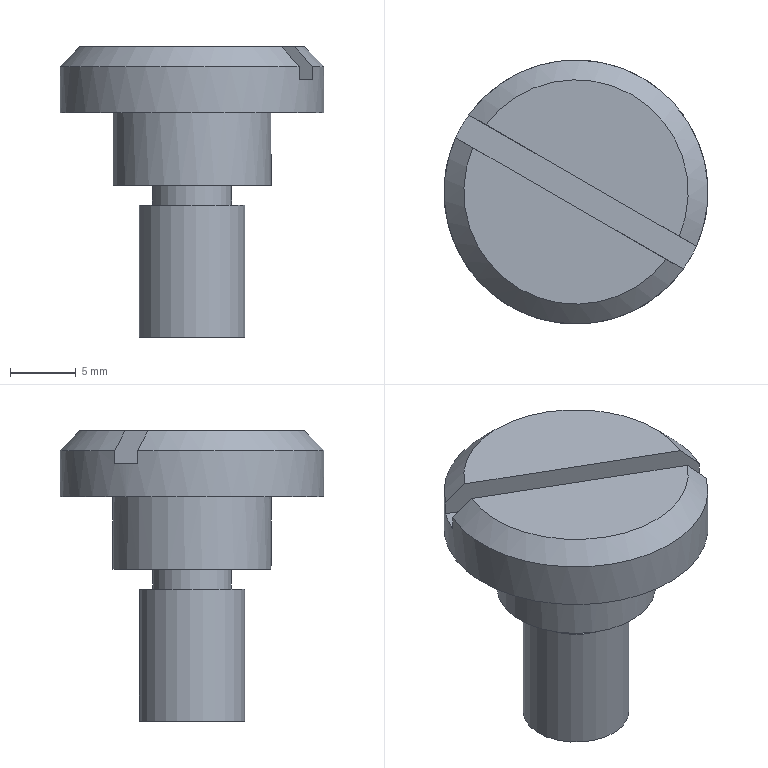Component | NX | DRILL_BUSH_SCREW | 1 solid | 15 faces | box 20 x 20 x 22 mm | volume 2575 mm3 | plane 9 | cylinder 4 | cone 2 | commonest cylinder face diameters 8 x1 6 x1 12 x1 20 x1
STEP:
#1=CARTESIAN_POINT('',(0.,0.,0.));
#2=DIRECTION('',(0.,0.,1.));
#3=DIRECTION('',(1.,0.,0.));
#4=AXIS2_PLACEMENT_3D('',#1,#2,#3);
#5=CARTESIAN_POINT('',(-19.19,-50.12,210.5));
#6=VERTEX_POINT('',#5);
#7=CARTESIAN_POINT('',(-33.81,-41.679,210.5));
#8=VERTEX_POINT('',#7);
#9=CARTESIAN_POINT('',(-13.077,-53.649,210.5));
#10=DIRECTION('',(-0.866,0.5,0.));
#11=VECTOR('',#10,1.);
#12=LINE('',#9,#11);
#13=CARTESIAN_POINT('',(-27.,-46.765,210.5));
#14=DIRECTION('',(0.,0.,1.));
#15=DIRECTION('',(-0.866,0.5,0.));
#16=AXIS2_PLACEMENT_3D('',#13,#14,#15);
#17=PLANE('',#16);
#18=CARTESIAN_POINT('',(-15.5,-1.));
#19=DIRECTION('',(1.,0.));
#20=VECTOR('',#19,1.);
#21=LINE('',#18,#20);
#22=(GEOMETRIC_REPRESENTATION_CONTEXT(2)PARAMETRIC_REPRESENTATION_CONTEXT()REPRESENTATION_CONTEXT('',''));
#23=DEFINITIONAL_REPRESENTATION('',(#21),#22);
#24=PCURVE('',#17,#23);
#25=CARTESIAN_POINT('',(-13.077,-53.649,208.));
#26=DIRECTION('',(0.5,0.866,0.));
#27=DIRECTION('',(0.,0.,-1.));
#28=AXIS2_PLACEMENT_3D('',#25,#26,#27);
#29=PLANE('',#28);
#30=CARTESIAN_POINT('',(-2.5,0.));
#31=DIRECTION('',(0.,1.));
#32=VECTOR('',#31,1.);
#33=LINE('',#30,#32);
#34=(GEOMETRIC_REPRESENTATION_CONTEXT(2)PARAMETRIC_REPRESENTATION_CONTEXT()REPRESENTATION_CONTEXT('',''));
#35=DEFINITIONAL_REPRESENTATION('',(#33),#34);
#36=PCURVE('',#29,#35);
#37=SURFACE_CURVE('',#12,(#24,#36),.PCURVE_S1.);
#38=EDGE_CURVE('',#6,#8,#37,.T.);
#39=ORIENTED_EDGE('',*,*,#38,.F.);
#40=CARTESIAN_POINT('',(-27.,-46.765,210.5));
#41=DIRECTION('',(0.,0.,1.));
#42=DIRECTION('',(-0.866,0.5,0.));
#43=AXIS2_PLACEMENT_3D('',#40,#41,#42);
#44=CIRCLE('',#43,8.5);
#45=CARTESIAN_POINT('',(0.,0.));
#46=DIRECTION('',(1.,0.));
#47=AXIS2_PLACEMENT_2D('',#45,#46);
#48=CIRCLE('',#47,8.5);
#49=(GEOMETRIC_REPRESENTATION_CONTEXT(2)PARAMETRIC_REPRESENTATION_CONTEXT()REPRESENTATION_CONTEXT('',''));
#50=DEFINITIONAL_REPRESENTATION('',(#48),#49);
#51=PCURVE('',#17,#50);
#52=CARTESIAN_POINT('',(-27.,-46.765,209.));
#53=DIRECTION('',(0.,0.,-1.));
#54=DIRECTION('',(0.866,-0.5,0.));
#55=AXIS2_PLACEMENT_3D('',#52,#53,#54);
#56=CONICAL_SURFACE('',#55,10.,0.7854);
#57=CARTESIAN_POINT('',(9.425,-1.5));
#58=DIRECTION('',(-1.,-0.));
#59=VECTOR('',#58,1.);
#60=LINE('',#57,#59);
#61=(GEOMETRIC_REPRESENTATION_CONTEXT(2)PARAMETRIC_REPRESENTATION_CONTEXT()REPRESENTATION_CONTEXT('',''));
#62=DEFINITIONAL_REPRESENTATION('',(#60),#61);
#63=PCURVE('',#56,#62);
#64=SURFACE_CURVE('',#44,(#51,#63),.PCURVE_S1.);
#65=EDGE_CURVE('',#6,#8,#64,.T.);
#66=ORIENTED_EDGE('',*,*,#65,.T.);
#67=EDGE_LOOP('',(#39,#66));
#68=FACE_BOUND('',#67,.T.);
#69=ADVANCED_FACE('',(#68),#17,.T.);
#70=CARTESIAN_POINT('',(-29.598,-45.265,198.5));
#71=VERTEX_POINT('',#70);
#72=CARTESIAN_POINT('',(-27.,-46.765,198.5));
#73=DIRECTION('',(0.,0.,1.));
#74=DIRECTION('',(-0.866,0.5,0.));
#75=AXIS2_PLACEMENT_3D('',#72,#73,#74);
#76=CIRCLE('',#75,3.);
#77=CARTESIAN_POINT('',(-27.,-46.765,198.5));
#78=DIRECTION('',(0.,0.,1.));
#79=DIRECTION('',(-0.866,0.5,0.));
#80=AXIS2_PLACEMENT_3D('',#77,#78,#79);
#81=PLANE('',#80);
#82=CARTESIAN_POINT('',(0.,0.));
#83=DIRECTION('',(1.,-0.));
#84=AXIS2_PLACEMENT_2D('',#82,#83);
#85=CIRCLE('',#84,3.);
#86=(GEOMETRIC_REPRESENTATION_CONTEXT(2)PARAMETRIC_REPRESENTATION_CONTEXT()REPRESENTATION_CONTEXT('',''));
#87=DEFINITIONAL_REPRESENTATION('',(#85),#86);
#88=PCURVE('',#81,#87);
#89=CARTESIAN_POINT('',(-27.,-46.765,198.5));
#90=DIRECTION('',(0.,0.,1.));
#91=DIRECTION('',(-0.866,0.5,0.));
#92=AXIS2_PLACEMENT_3D('',#89,#90,#91);
#93=CYLINDRICAL_SURFACE('',#92,3.);
#94=CARTESIAN_POINT('',(0.,0.));
#95=DIRECTION('',(1.,0.));
#96=VECTOR('',#95,1.);
#97=LINE('',#94,#96);
#98=(GEOMETRIC_REPRESENTATION_CONTEXT(2)PARAMETRIC_REPRESENTATION_CONTEXT()REPRESENTATION_CONTEXT('',''));
#99=DEFINITIONAL_REPRESENTATION('',(#97),#98);
#100=PCURVE('',#93,#99);
#101=SURFACE_CURVE('',#76,(#88,#100),.PCURVE_S1.);
#102=EDGE_CURVE('',#71,#71,#101,.T.);
#103=ORIENTED_EDGE('',*,*,#102,.F.);
#104=EDGE_LOOP('',(#103));
#105=FACE_BOUND('',#104,.T.);
#106=CARTESIAN_POINT('',(-30.464,-44.765,198.5));
#107=VERTEX_POINT('',#106);
#108=CARTESIAN_POINT('',(-27.,-46.765,198.5));
#109=DIRECTION('',(0.,0.,-1.));
#110=DIRECTION('',(-0.866,0.5,0.));
#111=AXIS2_PLACEMENT_3D('',#108,#109,#110);
#112=CIRCLE('',#111,4.);
#113=CARTESIAN_POINT('',(4.,-0.));
#114=CARTESIAN_POINT('',(4.,-6.928));
#115=CARTESIAN_POINT('',(-2.,-3.464));
#116=CARTESIAN_POINT('',(-8.,0.));
#117=CARTESIAN_POINT('',(-2.,3.464));
#118=CARTESIAN_POINT('',(4.,6.928));
#119=CARTESIAN_POINT('',(4.,-0.));
#120=(BOUNDED_CURVE()B_SPLINE_CURVE(2,(#113,#114,#115,#116,#117,#118,#119),.UNSPECIFIED.,.T.,.F.)B_SPLINE_CURVE_WITH_KNOTS((1,2,2,2,2,1),(-2.094,0.,2.094,4.189,6.283,8.378),.UNSPECIFIED.)CURVE()GEOMETRIC_REPRESENTATION_ITEM()RATIONAL_B_SPLINE_CURVE((1.,0.5,1.,0.5,1.,0.5,1.))REPRESENTATION_ITEM(''));
#121=(GEOMETRIC_REPRESENTATION_CONTEXT(2)PARAMETRIC_REPRESENTATION_CONTEXT()REPRESENTATION_CONTEXT('',''));
#122=DEFINITIONAL_REPRESENTATION('',(#120),#121);
#123=PCURVE('',#81,#122);
#124=CARTESIAN_POINT('',(-27.,-46.765,188.5));
#125=DIRECTION('',(0.,0.,1.));
#126=DIRECTION('',(-0.866,0.5,0.));
#127=AXIS2_PLACEMENT_3D('',#124,#125,#126);
#128=CYLINDRICAL_SURFACE('',#127,4.);
#129=CARTESIAN_POINT('',(6.283,10.));
#130=DIRECTION('',(-1.,0.));
#131=VECTOR('',#130,1.);
#132=LINE('',#129,#131);
#133=(GEOMETRIC_REPRESENTATION_CONTEXT(2)PARAMETRIC_REPRESENTATION_CONTEXT()REPRESENTATION_CONTEXT('',''));
#134=DEFINITIONAL_REPRESENTATION('',(#132),#133);
#135=PCURVE('',#128,#134);
#136=SURFACE_CURVE('',#112,(#123,#135),.PCURVE_S1.);
#137=EDGE_CURVE('',#107,#107,#136,.T.);
#138=ORIENTED_EDGE('',*,*,#137,.F.);
#139=EDGE_LOOP('',(#138));
#140=FACE_BOUND('',#139,.T.);
#141=ADVANCED_FACE('',(#105,#140),#81,.T.);
#142=CARTESIAN_POINT('',(-30.464,-44.765,188.5));
#143=VERTEX_POINT('',#142);
#144=CARTESIAN_POINT('',(-27.,-46.765,188.5));
#145=DIRECTION('',(0.,0.,1.));
#146=DIRECTION('',(-0.866,0.5,0.));
#147=AXIS2_PLACEMENT_3D('',#144,#145,#146);
#148=CIRCLE('',#147,4.);
#149=CARTESIAN_POINT('',(-27.,-46.765,188.5));
#150=DIRECTION('',(0.,0.,-1.));
#151=DIRECTION('',(0.866,-0.5,0.));
#152=AXIS2_PLACEMENT_3D('',#149,#150,#151);
#153=PLANE('',#152);
#154=CARTESIAN_POINT('',(-4.,-0.));
#155=CARTESIAN_POINT('',(-4.,6.928));
#156=CARTESIAN_POINT('',(2.,3.464));
#157=CARTESIAN_POINT('',(8.,0.));
#158=CARTESIAN_POINT('',(2.,-3.464));
#159=CARTESIAN_POINT('',(-4.,-6.928));
#160=CARTESIAN_POINT('',(-4.,-0.));
#161=(BOUNDED_CURVE()B_SPLINE_CURVE(2,(#154,#155,#156,#157,#158,#159,#160),.UNSPECIFIED.,.T.,.F.)B_SPLINE_CURVE_WITH_KNOTS((1,2,2,2,2,1),(-2.094,0.,2.094,4.189,6.283,8.378),.UNSPECIFIED.)CURVE()GEOMETRIC_REPRESENTATION_ITEM()RATIONAL_B_SPLINE_CURVE((1.,0.5,1.,0.5,1.,0.5,1.))REPRESENTATION_ITEM(''));
#162=(GEOMETRIC_REPRESENTATION_CONTEXT(2)PARAMETRIC_REPRESENTATION_CONTEXT()REPRESENTATION_CONTEXT('',''));
#163=DEFINITIONAL_REPRESENTATION('',(#161),#162);
#164=PCURVE('',#153,#163);
#165=CARTESIAN_POINT('',(0.,0.));
#166=DIRECTION('',(1.,0.));
#167=VECTOR('',#166,1.);
#168=LINE('',#165,#167);
#169=(GEOMETRIC_REPRESENTATION_CONTEXT(2)PARAMETRIC_REPRESENTATION_CONTEXT()REPRESENTATION_CONTEXT('',''));
#170=DEFINITIONAL_REPRESENTATION('',(#168),#169);
#171=PCURVE('',#128,#170);
#172=SURFACE_CURVE('',#148,(#164,#171),.PCURVE_S1.);
#173=EDGE_CURVE('',#143,#143,#172,.T.);
#174=ORIENTED_EDGE('',*,*,#173,.F.);
#175=EDGE_LOOP('',(#174));
#176=FACE_BOUND('',#175,.T.);
#177=ADVANCED_FACE('',(#176),#153,.T.);
#178=ORIENTED_EDGE('',*,*,#137,.T.);
#179=CARTESIAN_POINT('',(-30.464,-44.765,188.5));
#180=CARTESIAN_POINT('',(-30.464,-44.765,198.5));
#181=B_SPLINE_CURVE_WITH_KNOTS('',1,(#179,#180),.UNSPECIFIED.,.F.,.F.,(2,2),(0.,10.),.PIECEWISE_BEZIER_KNOTS.);
#182=CARTESIAN_POINT('',(0.,0.));
#183=DIRECTION('',(0.,1.));
#184=VECTOR('',#183,1.);
#185=LINE('',#182,#184);
#186=(GEOMETRIC_REPRESENTATION_CONTEXT(2)PARAMETRIC_REPRESENTATION_CONTEXT()REPRESENTATION_CONTEXT('',''));
#187=DEFINITIONAL_REPRESENTATION('',(#185),#186);
#188=PCURVE('',#128,#187);
#189=CARTESIAN_POINT('',(6.283,0.));
#190=DIRECTION('',(0.,1.));
#191=VECTOR('',#190,1.);
#192=LINE('',#189,#191);
#193=(GEOMETRIC_REPRESENTATION_CONTEXT(2)PARAMETRIC_REPRESENTATION_CONTEXT()REPRESENTATION_CONTEXT('',''));
#194=DEFINITIONAL_REPRESENTATION('',(#192),#193);
#195=PCURVE('',#128,#194);
#196=SEAM_CURVE('',#181,(#188,#195),.PCURVE_S1.);
#197=EDGE_CURVE('',#143,#107,#196,.T.);
#198=ORIENTED_EDGE('',*,*,#197,.F.);
#199=ORIENTED_EDGE('',*,*,#173,.T.);
#200=ORIENTED_EDGE('',*,*,#197,.T.);
#201=EDGE_LOOP('',(#178,#198,#199,#200));
#202=FACE_BOUND('',#201,.T.);
#203=ADVANCED_FACE('',(#202),#128,.T.);
#204=CARTESIAN_POINT('',(-29.598,-45.265,200.));
#205=VERTEX_POINT('',#204);
#206=CARTESIAN_POINT('',(-24.402,-48.265,200.));
#207=VERTEX_POINT('',#206);
#208=CARTESIAN_POINT('',(-27.,-46.765,200.));
#209=DIRECTION('',(0.,0.,1.));
#210=DIRECTION('',(0.866,-0.5,0.));
#211=AXIS2_PLACEMENT_3D('',#208,#209,#210);
#212=CIRCLE('',#211,3.);
#213=CARTESIAN_POINT('',(-3.142,1.5));
#214=DIRECTION('',(1.,0.));
#215=VECTOR('',#214,1.);
#216=LINE('',#213,#215);
#217=(GEOMETRIC_REPRESENTATION_CONTEXT(2)PARAMETRIC_REPRESENTATION_CONTEXT()REPRESENTATION_CONTEXT('',''));
#218=DEFINITIONAL_REPRESENTATION('',(#216),#217);
#219=PCURVE('',#93,#218);
#220=CARTESIAN_POINT('',(-27.,-46.765,200.));
#221=DIRECTION('',(0.,0.,-1.));
#222=DIRECTION('',(0.866,-0.5,0.));
#223=AXIS2_PLACEMENT_3D('',#220,#221,#222);
#224=PLANE('',#223);
#225=CARTESIAN_POINT('',(3.,0.));
#226=CARTESIAN_POINT('',(3.,-5.196));
#227=CARTESIAN_POINT('',(-1.5,-2.598));
#228=CARTESIAN_POINT('',(-6.,-0.));
#229=CARTESIAN_POINT('',(-1.5,2.598));
#230=CARTESIAN_POINT('',(3.,5.196));
#231=CARTESIAN_POINT('',(3.,0.));
#232=(BOUNDED_CURVE()B_SPLINE_CURVE(2,(#225,#226,#227,#228,#229,#230,#231),.UNSPECIFIED.,.T.,.F.)B_SPLINE_CURVE_WITH_KNOTS((1,2,2,2,2,1),(-2.094,0.,2.094,4.189,6.283,8.378),.UNSPECIFIED.)CURVE()GEOMETRIC_REPRESENTATION_ITEM()RATIONAL_B_SPLINE_CURVE((1.,0.5,1.,0.5,1.,0.5,1.))REPRESENTATION_ITEM(''));
#233=(GEOMETRIC_REPRESENTATION_CONTEXT(2)PARAMETRIC_REPRESENTATION_CONTEXT()REPRESENTATION_CONTEXT('',''));
#234=DEFINITIONAL_REPRESENTATION('',(#232),#233);
#235=PCURVE('',#224,#234);
#236=SURFACE_CURVE('',#212,(#219,#235),.PCURVE_S1.);
#237=EDGE_CURVE('',#205,#207,#236,.T.);
#238=ORIENTED_EDGE('',*,*,#237,.F.);
#239=CARTESIAN_POINT('',(-29.598,-45.265,198.5));
#240=CARTESIAN_POINT('',(-29.598,-45.265,200.));
#241=B_SPLINE_CURVE_WITH_KNOTS('',1,(#239,#240),.UNSPECIFIED.,.F.,.F.,(2,2),(0.,1.5),.PIECEWISE_BEZIER_KNOTS.);
#242=CARTESIAN_POINT('',(0.,0.));
#243=DIRECTION('',(0.,1.));
#244=VECTOR('',#243,1.);
#245=LINE('',#242,#244);
#246=(GEOMETRIC_REPRESENTATION_CONTEXT(2)PARAMETRIC_REPRESENTATION_CONTEXT()REPRESENTATION_CONTEXT('',''));
#247=DEFINITIONAL_REPRESENTATION('',(#245),#246);
#248=PCURVE('',#93,#247);
#249=CARTESIAN_POINT('',(6.283,0.));
#250=DIRECTION('',(0.,1.));
#251=VECTOR('',#250,1.);
#252=LINE('',#249,#251);
#253=(GEOMETRIC_REPRESENTATION_CONTEXT(2)PARAMETRIC_REPRESENTATION_CONTEXT()REPRESENTATION_CONTEXT('',''));
#254=DEFINITIONAL_REPRESENTATION('',(#252),#253);
#255=PCURVE('',#93,#254);
#256=SEAM_CURVE('',#241,(#248,#255),.PCURVE_S1.);
#257=EDGE_CURVE('',#71,#205,#256,.T.);
#258=ORIENTED_EDGE('',*,*,#257,.F.);
#259=ORIENTED_EDGE('',*,*,#102,.T.);
#260=ORIENTED_EDGE('',*,*,#257,.T.);
#261=CARTESIAN_POINT('',(-27.,-46.765,200.));
#262=DIRECTION('',(0.,0.,1.));
#263=DIRECTION('',(0.866,-0.5,0.));
#264=AXIS2_PLACEMENT_3D('',#261,#262,#263);
#265=CIRCLE('',#264,3.);
#266=CARTESIAN_POINT('',(3.142,1.5));
#267=DIRECTION('',(1.,0.));
#268=VECTOR('',#267,1.);
#269=LINE('',#266,#268);
#270=(GEOMETRIC_REPRESENTATION_CONTEXT(2)PARAMETRIC_REPRESENTATION_CONTEXT()REPRESENTATION_CONTEXT('',''));
#271=DEFINITIONAL_REPRESENTATION('',(#269),#270);
#272=PCURVE('',#93,#271);
#273=CARTESIAN_POINT('',(3.,0.));
#274=CARTESIAN_POINT('',(3.,-5.196));
#275=CARTESIAN_POINT('',(-1.5,-2.598));
#276=CARTESIAN_POINT('',(-6.,-0.));
#277=CARTESIAN_POINT('',(-1.5,2.598));
#278=CARTESIAN_POINT('',(3.,5.196));
#279=CARTESIAN_POINT('',(3.,0.));
#280=(BOUNDED_CURVE()B_SPLINE_CURVE(2,(#273,#274,#275,#276,#277,#278,#279),.UNSPECIFIED.,.T.,.F.)B_SPLINE_CURVE_WITH_KNOTS((1,2,2,2,2,1),(-2.094,0.,2.094,4.189,6.283,8.378),.UNSPECIFIED.)CURVE()GEOMETRIC_REPRESENTATION_ITEM()RATIONAL_B_SPLINE_CURVE((1.,0.5,1.,0.5,1.,0.5,1.))REPRESENTATION_ITEM(''));
#281=(GEOMETRIC_REPRESENTATION_CONTEXT(2)PARAMETRIC_REPRESENTATION_CONTEXT()REPRESENTATION_CONTEXT('',''));
#282=DEFINITIONAL_REPRESENTATION('',(#280),#281);
#283=PCURVE('',#224,#282);
#284=SURFACE_CURVE('',#265,(#272,#283),.PCURVE_S1.);
#285=EDGE_CURVE('',#207,#205,#284,.T.);
#286=ORIENTED_EDGE('',*,*,#285,.F.);
#287=EDGE_LOOP('',(#238,#258,#259,#260,#286));
#288=FACE_BOUND('',#287,.T.);
#289=ADVANCED_FACE('',(#288),#93,.T.);
#290=ORIENTED_EDGE('',*,*,#285,.T.);
#291=ORIENTED_EDGE('',*,*,#237,.T.);
#292=EDGE_LOOP('',(#290,#291));
#293=FACE_BOUND('',#292,.T.);
#294=CARTESIAN_POINT('',(-32.196,-43.765,200.));
#295=VERTEX_POINT('',#294);
#296=CARTESIAN_POINT('',(-27.,-46.765,200.));
#297=DIRECTION('',(0.,0.,1.));
#298=DIRECTION('',(-0.866,0.5,0.));
#299=AXIS2_PLACEMENT_3D('',#296,#297,#298);
#300=CIRCLE('',#299,6.);
#301=CARTESIAN_POINT('',(-6.,0.));
#302=CARTESIAN_POINT('',(-6.,10.392));
#303=CARTESIAN_POINT('',(3.,5.196));
#304=CARTESIAN_POINT('',(12.,0.));
#305=CARTESIAN_POINT('',(3.,-5.196));
#306=CARTESIAN_POINT('',(-6.,-10.392));
#307=CARTESIAN_POINT('',(-6.,0.));
#308=(BOUNDED_CURVE()B_SPLINE_CURVE(2,(#301,#302,#303,#304,#305,#306,#307),.UNSPECIFIED.,.T.,.F.)B_SPLINE_CURVE_WITH_KNOTS((1,2,2,2,2,1),(-2.094,0.,2.094,4.189,6.283,8.378),.UNSPECIFIED.)CURVE()GEOMETRIC_REPRESENTATION_ITEM()RATIONAL_B_SPLINE_CURVE((1.,0.5,1.,0.5,1.,0.5,1.))REPRESENTATION_ITEM(''));
#309=(GEOMETRIC_REPRESENTATION_CONTEXT(2)PARAMETRIC_REPRESENTATION_CONTEXT()REPRESENTATION_CONTEXT('',''));
#310=DEFINITIONAL_REPRESENTATION('',(#308),#309);
#311=PCURVE('',#224,#310);
#312=CARTESIAN_POINT('',(-27.,-46.765,200.));
#313=DIRECTION('',(0.,0.,1.));
#314=DIRECTION('',(-0.866,0.5,0.));
#315=AXIS2_PLACEMENT_3D('',#312,#313,#314);
#316=CYLINDRICAL_SURFACE('',#315,6.);
#317=CARTESIAN_POINT('',(0.,0.));
#318=DIRECTION('',(1.,0.));
#319=VECTOR('',#318,1.);
#320=LINE('',#317,#319);
#321=(GEOMETRIC_REPRESENTATION_CONTEXT(2)PARAMETRIC_REPRESENTATION_CONTEXT()REPRESENTATION_CONTEXT('',''));
#322=DEFINITIONAL_REPRESENTATION('',(#320),#321);
#323=PCURVE('',#316,#322);
#324=SURFACE_CURVE('',#300,(#311,#323),.PCURVE_S1.);
#325=EDGE_CURVE('',#295,#295,#324,.T.);
#326=ORIENTED_EDGE('',*,*,#325,.F.);
#327=EDGE_LOOP('',(#326));
#328=FACE_BOUND('',#327,.T.);
#329=ADVANCED_FACE('',(#293,#328),#224,.T.);
#330=CARTESIAN_POINT('',(-32.196,-43.765,205.5));
#331=VERTEX_POINT('',#330);
#332=CARTESIAN_POINT('',(-21.804,-49.765,205.5));
#333=VERTEX_POINT('',#332);
#334=CARTESIAN_POINT('',(-27.,-46.765,205.5));
#335=DIRECTION('',(0.,0.,1.));
#336=DIRECTION('',(0.866,-0.5,0.));
#337=AXIS2_PLACEMENT_3D('',#334,#335,#336);
#338=CIRCLE('',#337,6.);
#339=CARTESIAN_POINT('',(-3.142,5.5));
#340=DIRECTION('',(1.,0.));
#341=VECTOR('',#340,1.);
#342=LINE('',#339,#341);
#343=(GEOMETRIC_REPRESENTATION_CONTEXT(2)PARAMETRIC_REPRESENTATION_CONTEXT()REPRESENTATION_CONTEXT('',''));
#344=DEFINITIONAL_REPRESENTATION('',(#342),#343);
#345=PCURVE('',#316,#344);
#346=CARTESIAN_POINT('',(-27.,-46.765,205.5));
#347=DIRECTION('',(0.,0.,-1.));
#348=DIRECTION('',(0.866,-0.5,0.));
#349=AXIS2_PLACEMENT_3D('',#346,#347,#348);
#350=PLANE('',#349);
#351=CARTESIAN_POINT('',(6.,0.));
#352=CARTESIAN_POINT('',(6.,-10.392));
#353=CARTESIAN_POINT('',(-3.,-5.196));
#354=CARTESIAN_POINT('',(-12.,-0.));
#355=CARTESIAN_POINT('',(-3.,5.196));
#356=CARTESIAN_POINT('',(6.,10.392));
#357=CARTESIAN_POINT('',(6.,0.));
#358=(BOUNDED_CURVE()B_SPLINE_CURVE(2,(#351,#352,#353,#354,#355,#356,#357),.UNSPECIFIED.,.T.,.F.)B_SPLINE_CURVE_WITH_KNOTS((1,2,2,2,2,1),(-2.094,0.,2.094,4.189,6.283,8.378),.UNSPECIFIED.)CURVE()GEOMETRIC_REPRESENTATION_ITEM()RATIONAL_B_SPLINE_CURVE((1.,0.5,1.,0.5,1.,0.5,1.))REPRESENTATION_ITEM(''));
#359=(GEOMETRIC_REPRESENTATION_CONTEXT(2)PARAMETRIC_REPRESENTATION_CONTEXT()REPRESENTATION_CONTEXT('',''));
#360=DEFINITIONAL_REPRESENTATION('',(#358),#359);
#361=PCURVE('',#350,#360);
#362=SURFACE_CURVE('',#338,(#345,#361),.PCURVE_S1.);
#363=EDGE_CURVE('',#331,#333,#362,.T.);
#364=ORIENTED_EDGE('',*,*,#363,.F.);
#365=CARTESIAN_POINT('',(-32.196,-43.765,200.));
#366=CARTESIAN_POINT('',(-32.196,-43.765,205.5));
#367=B_SPLINE_CURVE_WITH_KNOTS('',1,(#365,#366),.UNSPECIFIED.,.F.,.F.,(2,2),(0.,5.5),.PIECEWISE_BEZIER_KNOTS.);
#368=CARTESIAN_POINT('',(0.,0.));
#369=DIRECTION('',(0.,1.));
#370=VECTOR('',#369,1.);
#371=LINE('',#368,#370);
#372=(GEOMETRIC_REPRESENTATION_CONTEXT(2)PARAMETRIC_REPRESENTATION_CONTEXT()REPRESENTATION_CONTEXT('',''));
#373=DEFINITIONAL_REPRESENTATION('',(#371),#372);
#374=PCURVE('',#316,#373);
#375=CARTESIAN_POINT('',(6.283,0.));
#376=DIRECTION('',(0.,1.));
#377=VECTOR('',#376,1.);
#378=LINE('',#375,#377);
#379=(GEOMETRIC_REPRESENTATION_CONTEXT(2)PARAMETRIC_REPRESENTATION_CONTEXT()REPRESENTATION_CONTEXT('',''));
#380=DEFINITIONAL_REPRESENTATION('',(#378),#379);
#381=PCURVE('',#316,#380);
#382=SEAM_CURVE('',#367,(#374,#381),.PCURVE_S1.);
#383=EDGE_CURVE('',#295,#331,#382,.T.);
#384=ORIENTED_EDGE('',*,*,#383,.F.);
#385=ORIENTED_EDGE('',*,*,#325,.T.);
#386=ORIENTED_EDGE('',*,*,#383,.T.);
#387=CARTESIAN_POINT('',(-27.,-46.765,205.5));
#388=DIRECTION('',(0.,0.,1.));
#389=DIRECTION('',(0.866,-0.5,0.));
#390=AXIS2_PLACEMENT_3D('',#387,#388,#389);
#391=CIRCLE('',#390,6.);
#392=CARTESIAN_POINT('',(3.142,5.5));
#393=DIRECTION('',(1.,0.));
#394=VECTOR('',#393,1.);
#395=LINE('',#392,#394);
#396=(GEOMETRIC_REPRESENTATION_CONTEXT(2)PARAMETRIC_REPRESENTATION_CONTEXT()REPRESENTATION_CONTEXT('',''));
#397=DEFINITIONAL_REPRESENTATION('',(#395),#396);
#398=PCURVE('',#316,#397);
#399=CARTESIAN_POINT('',(6.,0.));
#400=CARTESIAN_POINT('',(6.,-10.392));
#401=CARTESIAN_POINT('',(-3.,-5.196));
#402=CARTESIAN_POINT('',(-12.,-0.));
#403=CARTESIAN_POINT('',(-3.,5.196));
#404=CARTESIAN_POINT('',(6.,10.392));
#405=CARTESIAN_POINT('',(6.,0.));
#406=(BOUNDED_CURVE()B_SPLINE_CURVE(2,(#399,#400,#401,#402,#403,#404,#405),.UNSPECIFIED.,.T.,.F.)B_SPLINE_CURVE_WITH_KNOTS((1,2,2,2,2,1),(-2.094,0.,2.094,4.189,6.283,8.378),.UNSPECIFIED.)CURVE()GEOMETRIC_REPRESENTATION_ITEM()RATIONAL_B_SPLINE_CURVE((1.,0.5,1.,0.5,1.,0.5,1.))REPRESENTATION_ITEM(''));
#407=(GEOMETRIC_REPRESENTATION_CONTEXT(2)PARAMETRIC_REPRESENTATION_CONTEXT()REPRESENTATION_CONTEXT('',''));
#408=DEFINITIONAL_REPRESENTATION('',(#406),#407);
#409=PCURVE('',#350,#408);
#410=SURFACE_CURVE('',#391,(#398,#409),.PCURVE_S1.);
#411=EDGE_CURVE('',#333,#331,#410,.T.);
#412=ORIENTED_EDGE('',*,*,#411,.F.);
#413=EDGE_LOOP('',(#364,#384,#385,#386,#412));
#414=FACE_BOUND('',#413,.T.);
#415=ADVANCED_FACE('',(#414),#316,.T.);
#416=CARTESIAN_POINT('',(-34.81,-43.411,210.5));
#417=VERTEX_POINT('',#416);
#418=CARTESIAN_POINT('',(-20.19,-51.852,210.5));
#419=VERTEX_POINT('',#418);
#420=CARTESIAN_POINT('',(-40.923,-39.881,210.5));
#421=DIRECTION('',(0.866,-0.5,0.));
#422=VECTOR('',#421,1.);
#423=LINE('',#420,#422);
#424=CARTESIAN_POINT('',(-27.,-46.765,210.5));
#425=DIRECTION('',(0.,0.,1.));
#426=DIRECTION('',(-0.866,0.5,0.));
#427=AXIS2_PLACEMENT_3D('',#424,#425,#426);
#428=PLANE('',#427);
#429=CARTESIAN_POINT('',(15.5,1.));
#430=DIRECTION('',(-1.,0.));
#431=VECTOR('',#430,1.);
#432=LINE('',#429,#431);
#433=(GEOMETRIC_REPRESENTATION_CONTEXT(2)PARAMETRIC_REPRESENTATION_CONTEXT()REPRESENTATION_CONTEXT('',''));
#434=DEFINITIONAL_REPRESENTATION('',(#432),#433);
#435=PCURVE('',#428,#434);
#436=CARTESIAN_POINT('',(-40.923,-39.881,208.));
#437=DIRECTION('',(-0.5,-0.866,0.));
#438=DIRECTION('',(0.,0.,1.));
#439=AXIS2_PLACEMENT_3D('',#436,#437,#438);
#440=PLANE('',#439);
#441=CARTESIAN_POINT('',(2.5,0.));
#442=DIRECTION('',(0.,-1.));
#443=VECTOR('',#442,1.);
#444=LINE('',#441,#443);
#445=(GEOMETRIC_REPRESENTATION_CONTEXT(2)PARAMETRIC_REPRESENTATION_CONTEXT()REPRESENTATION_CONTEXT('',''));
#446=DEFINITIONAL_REPRESENTATION('',(#444),#445);
#447=PCURVE('',#440,#446);
#448=SURFACE_CURVE('',#423,(#435,#447),.PCURVE_S1.);
#449=EDGE_CURVE('',#417,#419,#448,.T.);
#450=ORIENTED_EDGE('',*,*,#449,.F.);
#451=CARTESIAN_POINT('',(-27.,-46.765,210.5));
#452=DIRECTION('',(0.,0.,1.));
#453=DIRECTION('',(-0.866,0.5,0.));
#454=AXIS2_PLACEMENT_3D('',#451,#452,#453);
#455=CIRCLE('',#454,8.5);
#456=CARTESIAN_POINT('',(0.,0.));
#457=DIRECTION('',(1.,0.));
#458=AXIS2_PLACEMENT_2D('',#456,#457);
#459=CIRCLE('',#458,8.5);
#460=(GEOMETRIC_REPRESENTATION_CONTEXT(2)PARAMETRIC_REPRESENTATION_CONTEXT()REPRESENTATION_CONTEXT('',''));
#461=DEFINITIONAL_REPRESENTATION('',(#459),#460);
#462=PCURVE('',#428,#461);
#463=CARTESIAN_POINT('',(-27.,-46.765,209.));
#464=DIRECTION('',(0.,0.,-1.));
#465=DIRECTION('',(0.866,-0.5,0.));
#466=AXIS2_PLACEMENT_3D('',#463,#464,#465);
#467=CONICAL_SURFACE('',#466,10.,0.7854);
#468=CARTESIAN_POINT('',(3.142,-1.5));
#469=DIRECTION('',(-1.,0.));
#470=VECTOR('',#469,1.);
#471=LINE('',#468,#470);
#472=(GEOMETRIC_REPRESENTATION_CONTEXT(2)PARAMETRIC_REPRESENTATION_CONTEXT()REPRESENTATION_CONTEXT('',''));
#473=DEFINITIONAL_REPRESENTATION('',(#471),#472);
#474=PCURVE('',#467,#473);
#475=SURFACE_CURVE('',#455,(#462,#474),.PCURVE_S1.);
#476=EDGE_CURVE('',#417,#419,#475,.T.);
#477=ORIENTED_EDGE('',*,*,#476,.T.);
#478=EDGE_LOOP('',(#450,#477));
#479=FACE_BOUND('',#478,.T.);
#480=ADVANCED_FACE('',(#479),#428,.T.);
#481=ORIENTED_EDGE('',*,*,#411,.T.);
#482=ORIENTED_EDGE('',*,*,#363,.T.);
#483=EDGE_LOOP('',(#481,#482));
#484=FACE_BOUND('',#483,.T.);
#485=CARTESIAN_POINT('',(-35.66,-41.765,205.5));
#486=VERTEX_POINT('',#485);
#487=CARTESIAN_POINT('',(-27.,-46.765,205.5));
#488=DIRECTION('',(0.,0.,1.));
#489=DIRECTION('',(-0.866,0.5,0.));
#490=AXIS2_PLACEMENT_3D('',#487,#488,#489);
#491=CIRCLE('',#490,10.);
#492=CARTESIAN_POINT('',(-10.,0.));
#493=CARTESIAN_POINT('',(-10.,17.321));
#494=CARTESIAN_POINT('',(5.,8.66));
#495=CARTESIAN_POINT('',(20.,0.));
#496=CARTESIAN_POINT('',(5.,-8.66));
#497=CARTESIAN_POINT('',(-10.,-17.321));
#498=CARTESIAN_POINT('',(-10.,0.));
#499=(BOUNDED_CURVE()B_SPLINE_CURVE(2,(#492,#493,#494,#495,#496,#497,#498),.UNSPECIFIED.,.T.,.F.)B_SPLINE_CURVE_WITH_KNOTS((1,2,2,2,2,1),(-2.094,0.,2.094,4.189,6.283,8.378),.UNSPECIFIED.)CURVE()GEOMETRIC_REPRESENTATION_ITEM()RATIONAL_B_SPLINE_CURVE((1.,0.5,1.,0.5,1.,0.5,1.))REPRESENTATION_ITEM(''));
#500=(GEOMETRIC_REPRESENTATION_CONTEXT(2)PARAMETRIC_REPRESENTATION_CONTEXT()REPRESENTATION_CONTEXT('',''));
#501=DEFINITIONAL_REPRESENTATION('',(#499),#500);
#502=PCURVE('',#350,#501);
#503=CARTESIAN_POINT('',(-27.,-46.765,205.5));
#504=DIRECTION('',(0.,0.,1.));
#505=DIRECTION('',(-0.866,0.5,0.));
#506=AXIS2_PLACEMENT_3D('',#503,#504,#505);
#507=CYLINDRICAL_SURFACE('',#506,10.);
#508=CARTESIAN_POINT('',(0.,0.));
#509=DIRECTION('',(1.,0.));
#510=VECTOR('',#509,1.);
#511=LINE('',#508,#510);
#512=(GEOMETRIC_REPRESENTATION_CONTEXT(2)PARAMETRIC_REPRESENTATION_CONTEXT()REPRESENTATION_CONTEXT('',''));
#513=DEFINITIONAL_REPRESENTATION('',(#511),#512);
#514=PCURVE('',#507,#513);
#515=SURFACE_CURVE('',#491,(#502,#514),.PCURVE_S1.);
#516=EDGE_CURVE('',#486,#486,#515,.T.);
#517=ORIENTED_EDGE('',*,*,#516,.F.);
#518=EDGE_LOOP('',(#517));
#519=FACE_BOUND('',#518,.T.);
#520=ADVANCED_FACE('',(#484,#519),#350,.T.);
#521=CARTESIAN_POINT('',(-35.117,-40.924,209.));
#522=VERTEX_POINT('',#521);
#523=CARTESIAN_POINT('',(-35.117,-40.924,208.));
#524=VERTEX_POINT('',#523);
#525=CARTESIAN_POINT('',(-35.117,-40.924,205.5));
#526=DIRECTION('',(0.,0.,-1.));
#527=VECTOR('',#526,1.);
#528=LINE('',#525,#527);
#529=CARTESIAN_POINT('',(6.183,0.));
#530=DIRECTION('',(0.,-1.));
#531=VECTOR('',#530,1.);
#532=LINE('',#529,#531);
#533=(GEOMETRIC_REPRESENTATION_CONTEXT(2)PARAMETRIC_REPRESENTATION_CONTEXT()REPRESENTATION_CONTEXT('',''));
#534=DEFINITIONAL_REPRESENTATION('',(#532),#533);
#535=PCURVE('',#507,#534);
#536=CARTESIAN_POINT('',(2.5,25.45));
#537=DIRECTION('',(1.,0.));
#538=VECTOR('',#537,1.);
#539=LINE('',#536,#538);
#540=(GEOMETRIC_REPRESENTATION_CONTEXT(2)PARAMETRIC_REPRESENTATION_CONTEXT()REPRESENTATION_CONTEXT('',''));
#541=DEFINITIONAL_REPRESENTATION('',(#539),#540);
#542=PCURVE('',#29,#541);
#543=SURFACE_CURVE('',#528,(#535,#542),.PCURVE_S1.);
#544=EDGE_CURVE('',#522,#524,#543,.T.);
#545=ORIENTED_EDGE('',*,*,#544,.F.);
#546=CARTESIAN_POINT('',(-17.883,-50.874,209.));
#547=VERTEX_POINT('',#546);
#548=CARTESIAN_POINT('',(-27.,-46.765,209.));
#549=DIRECTION('',(0.,0.,-1.));
#550=DIRECTION('',(-0.866,0.5,0.));
#551=AXIS2_PLACEMENT_3D('',#548,#549,#550);
#552=CIRCLE('',#551,10.);
#553=CARTESIAN_POINT('',(6.283,3.5));
#554=DIRECTION('',(-1.,0.));
#555=VECTOR('',#554,1.);
#556=LINE('',#553,#555);
#557=(GEOMETRIC_REPRESENTATION_CONTEXT(2)PARAMETRIC_REPRESENTATION_CONTEXT()REPRESENTATION_CONTEXT('',''));
#558=DEFINITIONAL_REPRESENTATION('',(#556),#557);
#559=PCURVE('',#507,#558);
#560=CARTESIAN_POINT('',(3.142,0.));
#561=DIRECTION('',(1.,0.));
#562=VECTOR('',#561,1.);
#563=LINE('',#560,#562);
#564=(GEOMETRIC_REPRESENTATION_CONTEXT(2)PARAMETRIC_REPRESENTATION_CONTEXT()REPRESENTATION_CONTEXT('',''));
#565=DEFINITIONAL_REPRESENTATION('',(#563),#564);
#566=PCURVE('',#56,#565);
#567=SURFACE_CURVE('',#552,(#559,#566),.PCURVE_S1.);
#568=EDGE_CURVE('',#522,#547,#567,.T.);
#569=ORIENTED_EDGE('',*,*,#568,.T.);
#570=CARTESIAN_POINT('',(-17.883,-50.874,208.));
#571=VERTEX_POINT('',#570);
#572=CARTESIAN_POINT('',(-17.883,-50.874,205.5));
#573=DIRECTION('',(0.,0.,1.));
#574=VECTOR('',#573,1.);
#575=LINE('',#572,#574);
#576=CARTESIAN_POINT('',(3.242,0.));
#577=DIRECTION('',(0.,1.));
#578=VECTOR('',#577,1.);
#579=LINE('',#576,#578);
#580=(GEOMETRIC_REPRESENTATION_CONTEXT(2)PARAMETRIC_REPRESENTATION_CONTEXT()REPRESENTATION_CONTEXT('',''));
#581=DEFINITIONAL_REPRESENTATION('',(#579),#580);
#582=PCURVE('',#507,#581);
#583=CARTESIAN_POINT('',(2.5,5.55));
#584=DIRECTION('',(-1.,0.));
#585=VECTOR('',#584,1.);
#586=LINE('',#583,#585);
#587=(GEOMETRIC_REPRESENTATION_CONTEXT(2)PARAMETRIC_REPRESENTATION_CONTEXT()REPRESENTATION_CONTEXT('',''));
#588=DEFINITIONAL_REPRESENTATION('',(#586),#587);
#589=PCURVE('',#29,#588);
#590=SURFACE_CURVE('',#575,(#582,#589),.PCURVE_S1.);
#591=EDGE_CURVE('',#571,#547,#590,.T.);
#592=ORIENTED_EDGE('',*,*,#591,.F.);
#593=CARTESIAN_POINT('',(-18.883,-52.606,208.));
#594=VERTEX_POINT('',#593);
#595=CARTESIAN_POINT('',(-27.,-46.765,208.));
#596=DIRECTION('',(0.,0.,-1.));
#597=DIRECTION('',(-0.866,0.5,0.));
#598=AXIS2_PLACEMENT_3D('',#595,#596,#597);
#599=CIRCLE('',#598,10.);
#600=CARTESIAN_POINT('',(6.283,2.5));
#601=DIRECTION('',(-1.,0.));
#602=VECTOR('',#601,1.);
#603=LINE('',#600,#602);
#604=(GEOMETRIC_REPRESENTATION_CONTEXT(2)PARAMETRIC_REPRESENTATION_CONTEXT()REPRESENTATION_CONTEXT('',''));
#605=DEFINITIONAL_REPRESENTATION('',(#603),#604);
#606=PCURVE('',#507,#605);
#607=CARTESIAN_POINT('',(-27.,-46.765,208.));
#608=DIRECTION('',(0.,0.,1.));
#609=DIRECTION('',(-0.866,0.5,0.));
#610=AXIS2_PLACEMENT_3D('',#607,#608,#609);
#611=PLANE('',#610);
#612=CARTESIAN_POINT('',(10.,0.));
#613=CARTESIAN_POINT('',(10.,-17.321));
#614=CARTESIAN_POINT('',(-5.,-8.66));
#615=CARTESIAN_POINT('',(-20.,-0.));
#616=CARTESIAN_POINT('',(-5.,8.66));
#617=CARTESIAN_POINT('',(10.,17.321));
#618=CARTESIAN_POINT('',(10.,0.));
#619=(BOUNDED_CURVE()B_SPLINE_CURVE(2,(#612,#613,#614,#615,#616,#617,#618),.UNSPECIFIED.,.T.,.F.)B_SPLINE_CURVE_WITH_KNOTS((1,2,2,2,2,1),(-2.094,0.,2.094,4.189,6.283,8.378),.UNSPECIFIED.)CURVE()GEOMETRIC_REPRESENTATION_ITEM()RATIONAL_B_SPLINE_CURVE((1.,0.5,1.,0.5,1.,0.5,1.))REPRESENTATION_ITEM(''));
#620=(GEOMETRIC_REPRESENTATION_CONTEXT(2)PARAMETRIC_REPRESENTATION_CONTEXT()REPRESENTATION_CONTEXT('',''));
#621=DEFINITIONAL_REPRESENTATION('',(#619),#620);
#622=PCURVE('',#611,#621);
#623=SURFACE_CURVE('',#599,(#606,#622),.PCURVE_S1.);
#624=EDGE_CURVE('',#571,#594,#623,.T.);
#625=ORIENTED_EDGE('',*,*,#624,.T.);
#626=CARTESIAN_POINT('',(-18.883,-52.606,209.));
#627=VERTEX_POINT('',#626);
#628=CARTESIAN_POINT('',(-18.883,-52.606,205.5));
#629=DIRECTION('',(0.,0.,-1.));
#630=VECTOR('',#629,1.);
#631=LINE('',#628,#630);
#632=CARTESIAN_POINT('',(3.041,0.));
#633=DIRECTION('',(0.,-1.));
#634=VECTOR('',#633,1.);
#635=LINE('',#632,#634);
#636=(GEOMETRIC_REPRESENTATION_CONTEXT(2)PARAMETRIC_REPRESENTATION_CONTEXT()REPRESENTATION_CONTEXT('',''));
#637=DEFINITIONAL_REPRESENTATION('',(#635),#636);
#638=PCURVE('',#507,#637);
#639=CARTESIAN_POINT('',(-2.5,-25.45));
#640=DIRECTION('',(-1.,0.));
#641=VECTOR('',#640,1.);
#642=LINE('',#639,#641);
#643=(GEOMETRIC_REPRESENTATION_CONTEXT(2)PARAMETRIC_REPRESENTATION_CONTEXT()REPRESENTATION_CONTEXT('',''));
#644=DEFINITIONAL_REPRESENTATION('',(#642),#643);
#645=PCURVE('',#440,#644);
#646=SURFACE_CURVE('',#631,(#638,#645),.PCURVE_S1.);
#647=EDGE_CURVE('',#627,#594,#646,.T.);
#648=ORIENTED_EDGE('',*,*,#647,.F.);
#649=CARTESIAN_POINT('',(-36.117,-42.656,209.));
#650=VERTEX_POINT('',#649);
#651=CARTESIAN_POINT('',(-27.,-46.765,209.));
#652=DIRECTION('',(0.,0.,-1.));
#653=DIRECTION('',(-0.866,0.5,0.));
#654=AXIS2_PLACEMENT_3D('',#651,#652,#653);
#655=CIRCLE('',#654,10.);
#656=CARTESIAN_POINT('',(6.283,3.5));
#657=DIRECTION('',(-1.,0.));
#658=VECTOR('',#657,1.);
#659=LINE('',#656,#658);
#660=(GEOMETRIC_REPRESENTATION_CONTEXT(2)PARAMETRIC_REPRESENTATION_CONTEXT()REPRESENTATION_CONTEXT('',''));
#661=DEFINITIONAL_REPRESENTATION('',(#659),#660);
#662=PCURVE('',#507,#661);
#663=CARTESIAN_POINT('',(-3.142,0.));
#664=DIRECTION('',(1.,-0.));
#665=VECTOR('',#664,1.);
#666=LINE('',#663,#665);
#667=(GEOMETRIC_REPRESENTATION_CONTEXT(2)PARAMETRIC_REPRESENTATION_CONTEXT()REPRESENTATION_CONTEXT('',''));
#668=DEFINITIONAL_REPRESENTATION('',(#666),#667);
#669=PCURVE('',#467,#668);
#670=SURFACE_CURVE('',#655,(#662,#669),.PCURVE_S1.);
#671=EDGE_CURVE('',#627,#650,#670,.T.);
#672=ORIENTED_EDGE('',*,*,#671,.T.);
#673=CARTESIAN_POINT('',(-36.117,-42.656,208.));
#674=VERTEX_POINT('',#673);
#675=CARTESIAN_POINT('',(-36.117,-42.656,205.5));
#676=DIRECTION('',(0.,0.,1.));
#677=VECTOR('',#676,1.);
#678=LINE('',#675,#677);
#679=CARTESIAN_POINT('',(0.1002,0.));
#680=DIRECTION('',(0.,1.));
#681=VECTOR('',#680,1.);
#682=LINE('',#679,#681);
#683=(GEOMETRIC_REPRESENTATION_CONTEXT(2)PARAMETRIC_REPRESENTATION_CONTEXT()REPRESENTATION_CONTEXT('',''));
#684=DEFINITIONAL_REPRESENTATION('',(#682),#683);
#685=PCURVE('',#507,#684);
#686=CARTESIAN_POINT('',(-2.5,-5.55));
#687=DIRECTION('',(1.,0.));
#688=VECTOR('',#687,1.);
#689=LINE('',#686,#688);
#690=(GEOMETRIC_REPRESENTATION_CONTEXT(2)PARAMETRIC_REPRESENTATION_CONTEXT()REPRESENTATION_CONTEXT('',''));
#691=DEFINITIONAL_REPRESENTATION('',(#689),#690);
#692=PCURVE('',#440,#691);
#693=SURFACE_CURVE('',#678,(#685,#692),.PCURVE_S1.);
#694=EDGE_CURVE('',#674,#650,#693,.T.);
#695=ORIENTED_EDGE('',*,*,#694,.F.);
#696=CARTESIAN_POINT('',(-35.66,-41.765,208.));
#697=VERTEX_POINT('',#696);
#698=CARTESIAN_POINT('',(-27.,-46.765,208.));
#699=DIRECTION('',(0.,0.,-1.));
#700=DIRECTION('',(-0.866,0.5,0.));
#701=AXIS2_PLACEMENT_3D('',#698,#699,#700);
#702=CIRCLE('',#701,10.);
#703=CARTESIAN_POINT('',(6.283,2.5));
#704=DIRECTION('',(-1.,0.));
#705=VECTOR('',#704,1.);
#706=LINE('',#703,#705);
#707=(GEOMETRIC_REPRESENTATION_CONTEXT(2)PARAMETRIC_REPRESENTATION_CONTEXT()REPRESENTATION_CONTEXT('',''));
#708=DEFINITIONAL_REPRESENTATION('',(#706),#707);
#709=PCURVE('',#507,#708);
#710=CARTESIAN_POINT('',(10.,0.));
#711=CARTESIAN_POINT('',(10.,-17.321));
#712=CARTESIAN_POINT('',(-5.,-8.66));
#713=CARTESIAN_POINT('',(-20.,-0.));
#714=CARTESIAN_POINT('',(-5.,8.66));
#715=CARTESIAN_POINT('',(10.,17.321));
#716=CARTESIAN_POINT('',(10.,0.));
#717=(BOUNDED_CURVE()B_SPLINE_CURVE(2,(#710,#711,#712,#713,#714,#715,#716),.UNSPECIFIED.,.T.,.F.)B_SPLINE_CURVE_WITH_KNOTS((1,2,2,2,2,1),(-2.094,0.,2.094,4.189,6.283,8.378),.UNSPECIFIED.)CURVE()GEOMETRIC_REPRESENTATION_ITEM()RATIONAL_B_SPLINE_CURVE((1.,0.5,1.,0.5,1.,0.5,1.))REPRESENTATION_ITEM(''));
#718=(GEOMETRIC_REPRESENTATION_CONTEXT(2)PARAMETRIC_REPRESENTATION_CONTEXT()REPRESENTATION_CONTEXT('',''));
#719=DEFINITIONAL_REPRESENTATION('',(#717),#718);
#720=PCURVE('',#611,#719);
#721=SURFACE_CURVE('',#702,(#709,#720),.PCURVE_S1.);
#722=EDGE_CURVE('',#674,#697,#721,.T.);
#723=ORIENTED_EDGE('',*,*,#722,.T.);
#724=CARTESIAN_POINT('',(-35.66,-41.765,205.5));
#725=CARTESIAN_POINT('',(-35.66,-41.765,208.));
#726=B_SPLINE_CURVE_WITH_KNOTS('',1,(#724,#725),.UNSPECIFIED.,.F.,.F.,(2,2),(0.,2.5),.PIECEWISE_BEZIER_KNOTS.);
#727=CARTESIAN_POINT('',(0.,0.));
#728=DIRECTION('',(0.,1.));
#729=VECTOR('',#728,1.);
#730=LINE('',#727,#729);
#731=(GEOMETRIC_REPRESENTATION_CONTEXT(2)PARAMETRIC_REPRESENTATION_CONTEXT()REPRESENTATION_CONTEXT('',''));
#732=DEFINITIONAL_REPRESENTATION('',(#730),#731);
#733=PCURVE('',#507,#732);
#734=CARTESIAN_POINT('',(6.283,0.));
#735=DIRECTION('',(0.,1.));
#736=VECTOR('',#735,1.);
#737=LINE('',#734,#736);
#738=(GEOMETRIC_REPRESENTATION_CONTEXT(2)PARAMETRIC_REPRESENTATION_CONTEXT()REPRESENTATION_CONTEXT('',''));
#739=DEFINITIONAL_REPRESENTATION('',(#737),#738);
#740=PCURVE('',#507,#739);
#741=SEAM_CURVE('',#726,(#733,#740),.PCURVE_S1.);
#742=EDGE_CURVE('',#486,#697,#741,.T.);
#743=ORIENTED_EDGE('',*,*,#742,.F.);
#744=ORIENTED_EDGE('',*,*,#516,.T.);
#745=ORIENTED_EDGE('',*,*,#742,.T.);
#746=CARTESIAN_POINT('',(-27.,-46.765,208.));
#747=DIRECTION('',(0.,0.,-1.));
#748=DIRECTION('',(-0.866,0.5,0.));
#749=AXIS2_PLACEMENT_3D('',#746,#747,#748);
#750=CIRCLE('',#749,10.);
#751=CARTESIAN_POINT('',(12.566,2.5));
#752=DIRECTION('',(-1.,0.));
#753=VECTOR('',#752,1.);
#754=LINE('',#751,#753);
#755=(GEOMETRIC_REPRESENTATION_CONTEXT(2)PARAMETRIC_REPRESENTATION_CONTEXT()REPRESENTATION_CONTEXT('',''));
#756=DEFINITIONAL_REPRESENTATION('',(#754),#755);
#757=PCURVE('',#507,#756);
#758=CARTESIAN_POINT('',(10.,0.));
#759=CARTESIAN_POINT('',(10.,-17.321));
#760=CARTESIAN_POINT('',(-5.,-8.66));
#761=CARTESIAN_POINT('',(-20.,-0.));
#762=CARTESIAN_POINT('',(-5.,8.66));
#763=CARTESIAN_POINT('',(10.,17.321));
#764=CARTESIAN_POINT('',(10.,0.));
#765=(BOUNDED_CURVE()B_SPLINE_CURVE(2,(#758,#759,#760,#761,#762,#763,#764),.UNSPECIFIED.,.T.,.F.)B_SPLINE_CURVE_WITH_KNOTS((1,2,2,2,2,1),(-2.094,0.,2.094,4.189,6.283,8.378),.UNSPECIFIED.)CURVE()GEOMETRIC_REPRESENTATION_ITEM()RATIONAL_B_SPLINE_CURVE((1.,0.5,1.,0.5,1.,0.5,1.))REPRESENTATION_ITEM(''));
#766=(GEOMETRIC_REPRESENTATION_CONTEXT(2)PARAMETRIC_REPRESENTATION_CONTEXT()REPRESENTATION_CONTEXT('',''));
#767=DEFINITIONAL_REPRESENTATION('',(#765),#766);
#768=PCURVE('',#611,#767);
#769=SURFACE_CURVE('',#750,(#757,#768),.PCURVE_S1.);
#770=EDGE_CURVE('',#697,#524,#769,.T.);
#771=ORIENTED_EDGE('',*,*,#770,.T.);
#772=EDGE_LOOP('',(#545,#569,#592,#625,#648,#672,#695,#723,#743,#744,#745,#771));
#773=FACE_BOUND('',#772,.T.);
#774=ADVANCED_FACE('',(#773),#507,.T.);
#775=ORIENTED_EDGE('',*,*,#591,.T.);
#776=CARTESIAN_POINT('',(-17.883,-50.874,209.));
#777=CARTESIAN_POINT('',(-18.319,-50.623,209.5));
#778=CARTESIAN_POINT('',(-18.754,-50.371,210.));
#779=CARTESIAN_POINT('',(-19.19,-50.12,210.5));
#780=B_SPLINE_CURVE_WITH_KNOTS('',3,(#776,#777,#778,#779),.UNSPECIFIED.,.F.,.F.,(4,4),(0.,1.),.PIECEWISE_BEZIER_KNOTS.);
#781=CARTESIAN_POINT('',(-1.,5.55));
#782=CARTESIAN_POINT('',(-1.5,6.053));
#783=CARTESIAN_POINT('',(-2.,6.556));
#784=CARTESIAN_POINT('',(-2.5,7.059));
#785=B_SPLINE_CURVE_WITH_KNOTS('',3,(#781,#782,#783,#784),.UNSPECIFIED.,.F.,.F.,(4,4),(0.,1.),.PIECEWISE_BEZIER_KNOTS.);
#786=(GEOMETRIC_REPRESENTATION_CONTEXT(2)PARAMETRIC_REPRESENTATION_CONTEXT()REPRESENTATION_CONTEXT('',''));
#787=DEFINITIONAL_REPRESENTATION('',(#785),#786);
#788=PCURVE('',#29,#787);
#789=CARTESIAN_POINT('',(6.183,0.));
#790=CARTESIAN_POINT('',(6.165,-1.5));
#791=B_SPLINE_CURVE_WITH_KNOTS('',1,(#789,#790),.UNSPECIFIED.,.F.,.F.,(2,2),(0.,1.),.PIECEWISE_BEZIER_KNOTS.);
#792=(GEOMETRIC_REPRESENTATION_CONTEXT(2)PARAMETRIC_REPRESENTATION_CONTEXT()REPRESENTATION_CONTEXT('',''));
#793=DEFINITIONAL_REPRESENTATION('',(#791),#792);
#794=PCURVE('',#56,#793);
#795=SURFACE_CURVE('',#780,(#788,#794),.PCURVE_S1.);
#796=EDGE_CURVE('',#547,#6,#795,.T.);
#797=ORIENTED_EDGE('',*,*,#796,.T.);
#798=ORIENTED_EDGE('',*,*,#38,.T.);
#799=CARTESIAN_POINT('',(-33.81,-41.679,210.5));
#800=CARTESIAN_POINT('',(-34.246,-41.427,210.));
#801=CARTESIAN_POINT('',(-34.681,-41.176,209.5));
#802=CARTESIAN_POINT('',(-35.117,-40.924,209.));
#803=B_SPLINE_CURVE_WITH_KNOTS('',3,(#799,#800,#801,#802),.UNSPECIFIED.,.F.,.F.,(4,4),(0.,1.),.PIECEWISE_BEZIER_KNOTS.);
#804=CARTESIAN_POINT('',(-2.5,23.941));
#805=CARTESIAN_POINT('',(-2.,24.444));
#806=CARTESIAN_POINT('',(-1.5,24.947));
#807=CARTESIAN_POINT('',(-1.,25.45));
#808=B_SPLINE_CURVE_WITH_KNOTS('',3,(#804,#805,#806,#807),.UNSPECIFIED.,.F.,.F.,(4,4),(0.,1.),.PIECEWISE_BEZIER_KNOTS.);
#809=(GEOMETRIC_REPRESENTATION_CONTEXT(2)PARAMETRIC_REPRESENTATION_CONTEXT()REPRESENTATION_CONTEXT('',''));
#810=DEFINITIONAL_REPRESENTATION('',(#808),#809);
#811=PCURVE('',#29,#810);
#812=CARTESIAN_POINT('',(3.26,-1.5));
#813=CARTESIAN_POINT('',(3.242,-0.));
#814=B_SPLINE_CURVE_WITH_KNOTS('',1,(#812,#813),.UNSPECIFIED.,.F.,.F.,(2,2),(0.,1.),.PIECEWISE_BEZIER_KNOTS.);
#815=(GEOMETRIC_REPRESENTATION_CONTEXT(2)PARAMETRIC_REPRESENTATION_CONTEXT()REPRESENTATION_CONTEXT('',''));
#816=DEFINITIONAL_REPRESENTATION('',(#814),#815);
#817=PCURVE('',#56,#816);
#818=SURFACE_CURVE('',#803,(#811,#817),.PCURVE_S1.);
#819=EDGE_CURVE('',#8,#522,#818,.T.);
#820=ORIENTED_EDGE('',*,*,#819,.T.);
#821=ORIENTED_EDGE('',*,*,#544,.T.);
#822=CARTESIAN_POINT('',(-13.077,-53.649,208.));
#823=DIRECTION('',(0.866,-0.5,0.));
#824=VECTOR('',#823,1.);
#825=LINE('',#822,#824);
#826=CARTESIAN_POINT('',(0.,0.));
#827=DIRECTION('',(0.,-1.));
#828=VECTOR('',#827,1.);
#829=LINE('',#826,#828);
#830=(GEOMETRIC_REPRESENTATION_CONTEXT(2)PARAMETRIC_REPRESENTATION_CONTEXT()REPRESENTATION_CONTEXT('',''));
#831=DEFINITIONAL_REPRESENTATION('',(#829),#830);
#832=PCURVE('',#29,#831);
#833=CARTESIAN_POINT('',(-15.5,-1.));
#834=DIRECTION('',(-1.,0.));
#835=VECTOR('',#834,1.);
#836=LINE('',#833,#835);
#837=(GEOMETRIC_REPRESENTATION_CONTEXT(2)PARAMETRIC_REPRESENTATION_CONTEXT()REPRESENTATION_CONTEXT('',''));
#838=DEFINITIONAL_REPRESENTATION('',(#836),#837);
#839=PCURVE('',#611,#838);
#840=SURFACE_CURVE('',#825,(#832,#839),.PCURVE_S1.);
#841=EDGE_CURVE('',#524,#571,#840,.T.);
#842=ORIENTED_EDGE('',*,*,#841,.T.);
#843=EDGE_LOOP('',(#775,#797,#798,#820,#821,#842));
#844=FACE_BOUND('',#843,.T.);
#845=ADVANCED_FACE('',(#844),#29,.F.);
#846=ORIENTED_EDGE('',*,*,#694,.T.);
#847=CARTESIAN_POINT('',(-36.117,-42.656,209.));
#848=CARTESIAN_POINT('',(-35.681,-42.908,209.5));
#849=CARTESIAN_POINT('',(-35.246,-43.159,210.));
#850=CARTESIAN_POINT('',(-34.81,-43.411,210.5));
#851=B_SPLINE_CURVE_WITH_KNOTS('',3,(#847,#848,#849,#850),.UNSPECIFIED.,.F.,.F.,(4,4),(0.,1.),.PIECEWISE_BEZIER_KNOTS.);
#852=CARTESIAN_POINT('',(1.,-5.55));
#853=CARTESIAN_POINT('',(1.5,-6.053));
#854=CARTESIAN_POINT('',(2.,-6.556));
#855=CARTESIAN_POINT('',(2.5,-7.059));
#856=B_SPLINE_CURVE_WITH_KNOTS('',3,(#852,#853,#854,#855),.UNSPECIFIED.,.F.,.F.,(4,4),(0.,1.),.PIECEWISE_BEZIER_KNOTS.);
#857=(GEOMETRIC_REPRESENTATION_CONTEXT(2)PARAMETRIC_REPRESENTATION_CONTEXT()REPRESENTATION_CONTEXT('',''));
#858=DEFINITIONAL_REPRESENTATION('',(#856),#857);
#859=PCURVE('',#440,#858);
#860=CARTESIAN_POINT('',(3.041,-0.));
#861=CARTESIAN_POINT('',(3.024,-1.5));
#862=B_SPLINE_CURVE_WITH_KNOTS('',1,(#860,#861),.UNSPECIFIED.,.F.,.F.,(2,2),(0.,1.),.PIECEWISE_BEZIER_KNOTS.);
#863=(GEOMETRIC_REPRESENTATION_CONTEXT(2)PARAMETRIC_REPRESENTATION_CONTEXT()REPRESENTATION_CONTEXT('',''));
#864=DEFINITIONAL_REPRESENTATION('',(#862),#863);
#865=PCURVE('',#467,#864);
#866=SURFACE_CURVE('',#851,(#859,#865),.PCURVE_S1.);
#867=EDGE_CURVE('',#650,#417,#866,.T.);
#868=ORIENTED_EDGE('',*,*,#867,.T.);
#869=ORIENTED_EDGE('',*,*,#449,.T.);
#870=CARTESIAN_POINT('',(-20.19,-51.852,210.5));
#871=CARTESIAN_POINT('',(-19.754,-52.103,210.));
#872=CARTESIAN_POINT('',(-19.319,-52.355,209.5));
#873=CARTESIAN_POINT('',(-18.883,-52.606,209.));
#874=B_SPLINE_CURVE_WITH_KNOTS('',3,(#870,#871,#872,#873),.UNSPECIFIED.,.F.,.F.,(4,4),(0.,1.),.PIECEWISE_BEZIER_KNOTS.);
#875=CARTESIAN_POINT('',(2.5,-23.941));
#876=CARTESIAN_POINT('',(2.,-24.444));
#877=CARTESIAN_POINT('',(1.5,-24.947));
#878=CARTESIAN_POINT('',(1.,-25.45));
#879=B_SPLINE_CURVE_WITH_KNOTS('',3,(#875,#876,#877,#878),.UNSPECIFIED.,.F.,.F.,(4,4),(0.,1.),.PIECEWISE_BEZIER_KNOTS.);
#880=(GEOMETRIC_REPRESENTATION_CONTEXT(2)PARAMETRIC_REPRESENTATION_CONTEXT()REPRESENTATION_CONTEXT('',''));
#881=DEFINITIONAL_REPRESENTATION('',(#879),#880);
#882=PCURVE('',#440,#881);
#883=CARTESIAN_POINT('',(0.1179,-1.5));
#884=CARTESIAN_POINT('',(0.1002,0.));
#885=B_SPLINE_CURVE_WITH_KNOTS('',1,(#883,#884),.UNSPECIFIED.,.F.,.F.,(2,2),(0.,1.),.PIECEWISE_BEZIER_KNOTS.);
#886=(GEOMETRIC_REPRESENTATION_CONTEXT(2)PARAMETRIC_REPRESENTATION_CONTEXT()REPRESENTATION_CONTEXT('',''));
#887=DEFINITIONAL_REPRESENTATION('',(#885),#886);
#888=PCURVE('',#467,#887);
#889=SURFACE_CURVE('',#874,(#882,#888),.PCURVE_S1.);
#890=EDGE_CURVE('',#419,#627,#889,.T.);
#891=ORIENTED_EDGE('',*,*,#890,.T.);
#892=ORIENTED_EDGE('',*,*,#647,.T.);
#893=CARTESIAN_POINT('',(-40.923,-39.881,208.));
#894=DIRECTION('',(-0.866,0.5,0.));
#895=VECTOR('',#894,1.);
#896=LINE('',#893,#895);
#897=CARTESIAN_POINT('',(0.,0.));
#898=DIRECTION('',(0.,1.));
#899=VECTOR('',#898,1.);
#900=LINE('',#897,#899);
#901=(GEOMETRIC_REPRESENTATION_CONTEXT(2)PARAMETRIC_REPRESENTATION_CONTEXT()REPRESENTATION_CONTEXT('',''));
#902=DEFINITIONAL_REPRESENTATION('',(#900),#901);
#903=PCURVE('',#440,#902);
#904=CARTESIAN_POINT('',(15.5,1.));
#905=DIRECTION('',(1.,0.));
#906=VECTOR('',#905,1.);
#907=LINE('',#904,#906);
#908=(GEOMETRIC_REPRESENTATION_CONTEXT(2)PARAMETRIC_REPRESENTATION_CONTEXT()REPRESENTATION_CONTEXT('',''));
#909=DEFINITIONAL_REPRESENTATION('',(#907),#908);
#910=PCURVE('',#611,#909);
#911=SURFACE_CURVE('',#896,(#903,#910),.PCURVE_S1.);
#912=EDGE_CURVE('',#594,#674,#911,.T.);
#913=ORIENTED_EDGE('',*,*,#912,.T.);
#914=EDGE_LOOP('',(#846,#868,#869,#891,#892,#913));
#915=FACE_BOUND('',#914,.T.);
#916=ADVANCED_FACE('',(#915),#440,.F.);
#917=ORIENTED_EDGE('',*,*,#841,.F.);
#918=ORIENTED_EDGE('',*,*,#770,.F.);
#919=ORIENTED_EDGE('',*,*,#722,.F.);
#920=ORIENTED_EDGE('',*,*,#912,.F.);
#921=ORIENTED_EDGE('',*,*,#624,.F.);
#922=EDGE_LOOP('',(#917,#918,#919,#920,#921));
#923=FACE_BOUND('',#922,.T.);
#924=ADVANCED_FACE('',(#923),#611,.T.);
#925=ORIENTED_EDGE('',*,*,#819,.F.);
#926=ORIENTED_EDGE('',*,*,#65,.F.);
#927=ORIENTED_EDGE('',*,*,#796,.F.);
#928=ORIENTED_EDGE('',*,*,#568,.F.);
#929=EDGE_LOOP('',(#925,#926,#927,#928));
#930=FACE_BOUND('',#929,.T.);
#931=ADVANCED_FACE('',(#930),#56,.T.);
#932=ORIENTED_EDGE('',*,*,#890,.F.);
#933=ORIENTED_EDGE('',*,*,#476,.F.);
#934=ORIENTED_EDGE('',*,*,#867,.F.);
#935=ORIENTED_EDGE('',*,*,#671,.F.);
#936=EDGE_LOOP('',(#932,#933,#934,#935));
#937=FACE_BOUND('',#936,.T.);
#938=ADVANCED_FACE('',(#937),#467,.T.);
#939=CLOSED_SHELL('',(#69,#141,#177,#203,#289,#329,#415,#480,#520,#774,#845,#916,#924,#931,#938));
#940=MANIFOLD_SOLID_BREP('',#939);
#941=(LENGTH_UNIT()NAMED_UNIT(*)SI_UNIT(.MILLI.,.METRE.));
#942=UNCERTAINTY_MEASURE_WITH_UNIT(LENGTH_MEASURE(0.002),#941,'','');
#943=(NAMED_UNIT(*)PLANE_ANGLE_UNIT()SI_UNIT($,.RADIAN.));
#944=(NAMED_UNIT(*)SI_UNIT($,.STERADIAN.)SOLID_ANGLE_UNIT());
#945=(GEOMETRIC_REPRESENTATION_CONTEXT(3)GLOBAL_UNCERTAINTY_ASSIGNED_CONTEXT((#942))GLOBAL_UNIT_ASSIGNED_CONTEXT((#941,#943,#944))REPRESENTATION_CONTEXT('',''));
#946=ADVANCED_BREP_SHAPE_REPRESENTATION('',(#4,#940),#945);